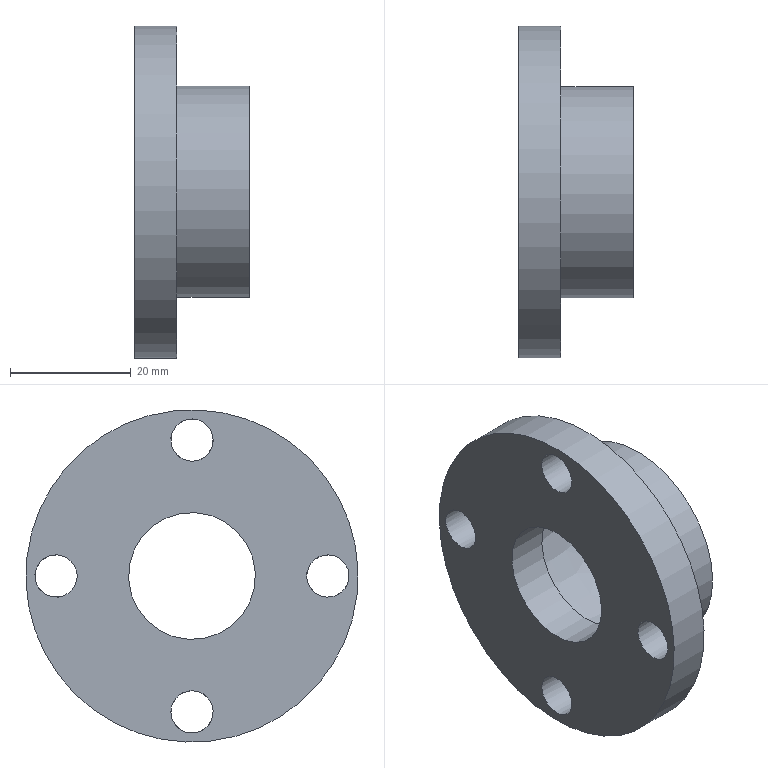Component | NX | BEARING_END_CAP_3 | 1 solid | 12 faces | box 19 x 55 x 55 mm | volume 16797 mm3 | cylinder 7 | plane 4 | cone 1 | commonest cylinder face diameters 7 x4 21 x1 35 x1 55 x1
STEP:
#1=CARTESIAN_POINT('',(0.,0.,0.));
#2=DIRECTION('',(0.,0.,1.));
#3=DIRECTION('',(1.,0.,0.));
#4=AXIS2_PLACEMENT_3D('',#1,#2,#3);
#5=CARTESIAN_POINT('',(407.689,-153.802,-1550.5));
#6=VERTEX_POINT('',#5);
#7=CARTESIAN_POINT('',(407.689,-152.777,-1548.025));
#8=VERTEX_POINT('',#7);
#9=CARTESIAN_POINT('',(407.689,-150.302,-1550.5));
#10=DIRECTION('',(-1.,0.,0.));
#11=DIRECTION('',(0.,-1.,0.));
#12=AXIS2_PLACEMENT_3D('',#9,#10,#11);
#13=CIRCLE('',#12,3.5);
#14=CARTESIAN_POINT('',(407.689,-169.747,-1553.555));
#15=DIRECTION('',(1.,0.,0.));
#16=DIRECTION('',(0.,0.7071,-0.7071));
#17=AXIS2_PLACEMENT_3D('',#14,#15,#16);
#18=PLANE('',#17);
#19=CARTESIAN_POINT('',(9.115,13.435));
#20=CARTESIAN_POINT('',(4.829,17.722));
#21=CARTESIAN_POINT('',(10.684,19.291));
#22=CARTESIAN_POINT('',(16.54,20.86));
#23=CARTESIAN_POINT('',(14.971,15.004));
#24=CARTESIAN_POINT('',(13.402,9.148));
#25=CARTESIAN_POINT('',(9.115,13.435));
#26=(BOUNDED_CURVE()B_SPLINE_CURVE(2,(#19,#20,#21,#22,#23,#24,#25),.UNSPECIFIED.,.T.,.F.)B_SPLINE_CURVE_WITH_KNOTS((1,2,2,2,2,1),(-2.094,0.,2.094,4.189,6.283,8.378),.UNSPECIFIED.)CURVE()GEOMETRIC_REPRESENTATION_ITEM()RATIONAL_B_SPLINE_CURVE((1.,0.5,1.,0.5,1.,0.5,1.))REPRESENTATION_ITEM(''));
#27=(GEOMETRIC_REPRESENTATION_CONTEXT(2)PARAMETRIC_REPRESENTATION_CONTEXT()REPRESENTATION_CONTEXT('',''));
#28=DEFINITIONAL_REPRESENTATION('',(#26),#27);
#29=PCURVE('',#18,#28);
#30=CARTESIAN_POINT('',(430.689,-150.302,-1550.5));
#31=DIRECTION('',(-1.,0.,0.));
#32=DIRECTION('',(0.,-0.7071,0.7071));
#33=AXIS2_PLACEMENT_3D('',#30,#31,#32);
#34=CYLINDRICAL_SURFACE('',#33,3.5);
#35=CARTESIAN_POINT('',(5.498,23.));
#36=DIRECTION('',(1.,0.));
#37=VECTOR('',#36,1.);
#38=LINE('',#35,#37);
#39=(GEOMETRIC_REPRESENTATION_CONTEXT(2)PARAMETRIC_REPRESENTATION_CONTEXT()REPRESENTATION_CONTEXT('',''));
#40=DEFINITIONAL_REPRESENTATION('',(#38),#39);
#41=PCURVE('',#34,#40);
#42=SURFACE_CURVE('',#13,(#29,#41),.PCURVE_S1.);
#43=EDGE_CURVE('',#6,#8,#42,.T.);
#44=ORIENTED_EDGE('',*,*,#43,.F.);
#45=CARTESIAN_POINT('',(407.689,-150.302,-1550.5));
#46=DIRECTION('',(-1.,0.,0.));
#47=DIRECTION('',(0.,-1.,0.));
#48=AXIS2_PLACEMENT_3D('',#45,#46,#47);
#49=CIRCLE('',#48,3.5);
#50=CARTESIAN_POINT('',(9.115,13.435));
#51=CARTESIAN_POINT('',(4.829,17.722));
#52=CARTESIAN_POINT('',(10.684,19.291));
#53=CARTESIAN_POINT('',(16.54,20.86));
#54=CARTESIAN_POINT('',(14.971,15.004));
#55=CARTESIAN_POINT('',(13.402,9.148));
#56=CARTESIAN_POINT('',(9.115,13.435));
#57=(BOUNDED_CURVE()B_SPLINE_CURVE(2,(#50,#51,#52,#53,#54,#55,#56),.UNSPECIFIED.,.T.,.F.)B_SPLINE_CURVE_WITH_KNOTS((1,2,2,2,2,1),(-2.094,0.,2.094,4.189,6.283,8.378),.UNSPECIFIED.)CURVE()GEOMETRIC_REPRESENTATION_ITEM()RATIONAL_B_SPLINE_CURVE((1.,0.5,1.,0.5,1.,0.5,1.))REPRESENTATION_ITEM(''));
#58=(GEOMETRIC_REPRESENTATION_CONTEXT(2)PARAMETRIC_REPRESENTATION_CONTEXT()REPRESENTATION_CONTEXT('',''));
#59=DEFINITIONAL_REPRESENTATION('',(#57),#58);
#60=PCURVE('',#18,#59);
#61=CARTESIAN_POINT('',(-0.7854,23.));
#62=DIRECTION('',(1.,0.));
#63=VECTOR('',#62,1.);
#64=LINE('',#61,#63);
#65=(GEOMETRIC_REPRESENTATION_CONTEXT(2)PARAMETRIC_REPRESENTATION_CONTEXT()REPRESENTATION_CONTEXT('',''));
#66=DEFINITIONAL_REPRESENTATION('',(#64),#65);
#67=PCURVE('',#34,#66);
#68=SURFACE_CURVE('',#49,(#60,#67),.PCURVE_S1.);
#69=EDGE_CURVE('',#8,#6,#68,.T.);
#70=ORIENTED_EDGE('',*,*,#69,.F.);
#71=EDGE_LOOP('',(#44,#70));
#72=FACE_BOUND('',#71,.T.);
#73=CARTESIAN_POINT('',(407.689,-172.802,-1576.5));
#74=VERTEX_POINT('',#73);
#75=CARTESIAN_POINT('',(407.689,-175.277,-1570.525));
#76=VERTEX_POINT('',#75);
#77=CARTESIAN_POINT('',(407.689,-172.802,-1573.));
#78=DIRECTION('',(-1.,0.,0.));
#79=DIRECTION('',(0.,0.,-1.));
#80=AXIS2_PLACEMENT_3D('',#77,#78,#79);
#81=CIRCLE('',#80,3.5);
#82=CARTESIAN_POINT('',(14.065,-18.385));
#83=CARTESIAN_POINT('',(9.778,-22.671));
#84=CARTESIAN_POINT('',(8.209,-16.816));
#85=CARTESIAN_POINT('',(6.64,-10.96));
#86=CARTESIAN_POINT('',(12.496,-12.529));
#87=CARTESIAN_POINT('',(18.352,-14.098));
#88=CARTESIAN_POINT('',(14.065,-18.385));
#89=(BOUNDED_CURVE()B_SPLINE_CURVE(2,(#82,#83,#84,#85,#86,#87,#88),.UNSPECIFIED.,.T.,.F.)B_SPLINE_CURVE_WITH_KNOTS((1,2,2,2,2,1),(-2.094,0.,2.094,4.189,6.283,8.378),.UNSPECIFIED.)CURVE()GEOMETRIC_REPRESENTATION_ITEM()RATIONAL_B_SPLINE_CURVE((1.,0.5,1.,0.5,1.,0.5,1.))REPRESENTATION_ITEM(''));
#90=(GEOMETRIC_REPRESENTATION_CONTEXT(2)PARAMETRIC_REPRESENTATION_CONTEXT()REPRESENTATION_CONTEXT('',''));
#91=DEFINITIONAL_REPRESENTATION('',(#89),#90);
#92=PCURVE('',#18,#91);
#93=CARTESIAN_POINT('',(430.689,-172.802,-1573.));
#94=DIRECTION('',(-1.,0.,0.));
#95=DIRECTION('',(0.,-0.7071,0.7071));
#96=AXIS2_PLACEMENT_3D('',#93,#94,#95);
#97=CYLINDRICAL_SURFACE('',#96,3.5);
#98=CARTESIAN_POINT('',(3.927,23.));
#99=DIRECTION('',(1.,0.));
#100=VECTOR('',#99,1.);
#101=LINE('',#98,#100);
#102=(GEOMETRIC_REPRESENTATION_CONTEXT(2)PARAMETRIC_REPRESENTATION_CONTEXT()REPRESENTATION_CONTEXT('',''));
#103=DEFINITIONAL_REPRESENTATION('',(#101),#102);
#104=PCURVE('',#97,#103);
#105=SURFACE_CURVE('',#81,(#92,#104),.PCURVE_S1.);
#106=EDGE_CURVE('',#74,#76,#105,.T.);
#107=ORIENTED_EDGE('',*,*,#106,.F.);
#108=CARTESIAN_POINT('',(407.689,-172.802,-1573.));
#109=DIRECTION('',(-1.,0.,0.));
#110=DIRECTION('',(0.,0.,-1.));
#111=AXIS2_PLACEMENT_3D('',#108,#109,#110);
#112=CIRCLE('',#111,3.5);
#113=CARTESIAN_POINT('',(14.065,-18.385));
#114=CARTESIAN_POINT('',(9.778,-22.671));
#115=CARTESIAN_POINT('',(8.209,-16.816));
#116=CARTESIAN_POINT('',(6.64,-10.96));
#117=CARTESIAN_POINT('',(12.496,-12.529));
#118=CARTESIAN_POINT('',(18.352,-14.098));
#119=CARTESIAN_POINT('',(14.065,-18.385));
#120=(BOUNDED_CURVE()B_SPLINE_CURVE(2,(#113,#114,#115,#116,#117,#118,#119),.UNSPECIFIED.,.T.,.F.)B_SPLINE_CURVE_WITH_KNOTS((1,2,2,2,2,1),(-2.094,0.,2.094,4.189,6.283,8.378),.UNSPECIFIED.)CURVE()GEOMETRIC_REPRESENTATION_ITEM()RATIONAL_B_SPLINE_CURVE((1.,0.5,1.,0.5,1.,0.5,1.))REPRESENTATION_ITEM(''));
#121=(GEOMETRIC_REPRESENTATION_CONTEXT(2)PARAMETRIC_REPRESENTATION_CONTEXT()REPRESENTATION_CONTEXT('',''));
#122=DEFINITIONAL_REPRESENTATION('',(#120),#121);
#123=PCURVE('',#18,#122);
#124=CARTESIAN_POINT('',(-2.356,23.));
#125=DIRECTION('',(1.,0.));
#126=VECTOR('',#125,1.);
#127=LINE('',#124,#126);
#128=(GEOMETRIC_REPRESENTATION_CONTEXT(2)PARAMETRIC_REPRESENTATION_CONTEXT()REPRESENTATION_CONTEXT('',''));
#129=DEFINITIONAL_REPRESENTATION('',(#127),#128);
#130=PCURVE('',#97,#129);
#131=SURFACE_CURVE('',#112,(#123,#130),.PCURVE_S1.);
#132=EDGE_CURVE('',#76,#74,#131,.T.);
#133=ORIENTED_EDGE('',*,*,#132,.F.);
#134=EDGE_LOOP('',(#107,#133));
#135=FACE_BOUND('',#134,.T.);
#136=CARTESIAN_POINT('',(407.689,-146.802,-1595.5));
#137=VERTEX_POINT('',#136);
#138=CARTESIAN_POINT('',(407.689,-152.777,-1593.025));
#139=VERTEX_POINT('',#138);
#140=CARTESIAN_POINT('',(407.689,-150.302,-1595.5));
#141=DIRECTION('',(-1.,0.,0.));
#142=DIRECTION('',(0.,1.,0.));
#143=AXIS2_PLACEMENT_3D('',#140,#141,#142);
#144=CIRCLE('',#143,3.5);
#145=CARTESIAN_POINT('',(45.885,-13.435));
#146=CARTESIAN_POINT('',(50.171,-17.722));
#147=CARTESIAN_POINT('',(44.316,-19.291));
#148=CARTESIAN_POINT('',(38.46,-20.86));
#149=CARTESIAN_POINT('',(40.029,-15.004));
#150=CARTESIAN_POINT('',(41.598,-9.148));
#151=CARTESIAN_POINT('',(45.885,-13.435));
#152=(BOUNDED_CURVE()B_SPLINE_CURVE(2,(#145,#146,#147,#148,#149,#150,#151),.UNSPECIFIED.,.T.,.F.)B_SPLINE_CURVE_WITH_KNOTS((1,2,2,2,2,1),(-2.094,0.,2.094,4.189,6.283,8.378),.UNSPECIFIED.)CURVE()GEOMETRIC_REPRESENTATION_ITEM()RATIONAL_B_SPLINE_CURVE((1.,0.5,1.,0.5,1.,0.5,1.))REPRESENTATION_ITEM(''));
#153=(GEOMETRIC_REPRESENTATION_CONTEXT(2)PARAMETRIC_REPRESENTATION_CONTEXT()REPRESENTATION_CONTEXT('',''));
#154=DEFINITIONAL_REPRESENTATION('',(#152),#153);
#155=PCURVE('',#18,#154);
#156=CARTESIAN_POINT('',(430.689,-150.302,-1595.5));
#157=DIRECTION('',(-1.,0.,0.));
#158=DIRECTION('',(0.,-0.7071,0.7071));
#159=AXIS2_PLACEMENT_3D('',#156,#157,#158);
#160=CYLINDRICAL_SURFACE('',#159,3.5);
#161=CARTESIAN_POINT('',(2.356,23.));
#162=DIRECTION('',(1.,0.));
#163=VECTOR('',#162,1.);
#164=LINE('',#161,#163);
#165=(GEOMETRIC_REPRESENTATION_CONTEXT(2)PARAMETRIC_REPRESENTATION_CONTEXT()REPRESENTATION_CONTEXT('',''));
#166=DEFINITIONAL_REPRESENTATION('',(#164),#165);
#167=PCURVE('',#160,#166);
#168=SURFACE_CURVE('',#144,(#155,#167),.PCURVE_S1.);
#169=EDGE_CURVE('',#137,#139,#168,.T.);
#170=ORIENTED_EDGE('',*,*,#169,.F.);
#171=CARTESIAN_POINT('',(407.689,-150.302,-1595.5));
#172=DIRECTION('',(-1.,0.,0.));
#173=DIRECTION('',(0.,1.,0.));
#174=AXIS2_PLACEMENT_3D('',#171,#172,#173);
#175=CIRCLE('',#174,3.5);
#176=CARTESIAN_POINT('',(45.885,-13.435));
#177=CARTESIAN_POINT('',(50.171,-17.722));
#178=CARTESIAN_POINT('',(44.316,-19.291));
#179=CARTESIAN_POINT('',(38.46,-20.86));
#180=CARTESIAN_POINT('',(40.029,-15.004));
#181=CARTESIAN_POINT('',(41.598,-9.148));
#182=CARTESIAN_POINT('',(45.885,-13.435));
#183=(BOUNDED_CURVE()B_SPLINE_CURVE(2,(#176,#177,#178,#179,#180,#181,#182),.UNSPECIFIED.,.T.,.F.)B_SPLINE_CURVE_WITH_KNOTS((1,2,2,2,2,1),(-2.094,0.,2.094,4.189,6.283,8.378),.UNSPECIFIED.)CURVE()GEOMETRIC_REPRESENTATION_ITEM()RATIONAL_B_SPLINE_CURVE((1.,0.5,1.,0.5,1.,0.5,1.))REPRESENTATION_ITEM(''));
#184=(GEOMETRIC_REPRESENTATION_CONTEXT(2)PARAMETRIC_REPRESENTATION_CONTEXT()REPRESENTATION_CONTEXT('',''));
#185=DEFINITIONAL_REPRESENTATION('',(#183),#184);
#186=PCURVE('',#18,#185);
#187=CARTESIAN_POINT('',(-3.927,23.));
#188=DIRECTION('',(1.,0.));
#189=VECTOR('',#188,1.);
#190=LINE('',#187,#189);
#191=(GEOMETRIC_REPRESENTATION_CONTEXT(2)PARAMETRIC_REPRESENTATION_CONTEXT()REPRESENTATION_CONTEXT('',''));
#192=DEFINITIONAL_REPRESENTATION('',(#190),#191);
#193=PCURVE('',#160,#192);
#194=SURFACE_CURVE('',#175,(#186,#193),.PCURVE_S1.);
#195=EDGE_CURVE('',#139,#137,#194,.T.);
#196=ORIENTED_EDGE('',*,*,#195,.F.);
#197=EDGE_LOOP('',(#170,#196));
#198=FACE_BOUND('',#197,.T.);
#199=CARTESIAN_POINT('',(407.689,-127.802,-1569.5));
#200=VERTEX_POINT('',#199);
#201=CARTESIAN_POINT('',(407.689,-130.277,-1570.525));
#202=VERTEX_POINT('',#201);
#203=CARTESIAN_POINT('',(407.689,-127.802,-1573.));
#204=DIRECTION('',(-1.,0.,0.));
#205=DIRECTION('',(0.,0.,1.));
#206=AXIS2_PLACEMENT_3D('',#203,#204,#205);
#207=CIRCLE('',#206,3.5);
#208=CARTESIAN_POINT('',(40.935,18.385));
#209=CARTESIAN_POINT('',(45.222,22.671));
#210=CARTESIAN_POINT('',(46.791,16.816));
#211=CARTESIAN_POINT('',(48.36,10.96));
#212=CARTESIAN_POINT('',(42.504,12.529));
#213=CARTESIAN_POINT('',(36.648,14.098));
#214=CARTESIAN_POINT('',(40.935,18.385));
#215=(BOUNDED_CURVE()B_SPLINE_CURVE(2,(#208,#209,#210,#211,#212,#213,#214),.UNSPECIFIED.,.T.,.F.)B_SPLINE_CURVE_WITH_KNOTS((1,2,2,2,2,1),(-2.094,0.,2.094,4.189,6.283,8.378),.UNSPECIFIED.)CURVE()GEOMETRIC_REPRESENTATION_ITEM()RATIONAL_B_SPLINE_CURVE((1.,0.5,1.,0.5,1.,0.5,1.))REPRESENTATION_ITEM(''));
#216=(GEOMETRIC_REPRESENTATION_CONTEXT(2)PARAMETRIC_REPRESENTATION_CONTEXT()REPRESENTATION_CONTEXT('',''));
#217=DEFINITIONAL_REPRESENTATION('',(#215),#216);
#218=PCURVE('',#18,#217);
#219=CARTESIAN_POINT('',(430.689,-127.802,-1573.));
#220=DIRECTION('',(-1.,0.,0.));
#221=DIRECTION('',(0.,-0.7071,0.7071));
#222=AXIS2_PLACEMENT_3D('',#219,#220,#221);
#223=CYLINDRICAL_SURFACE('',#222,3.5);
#224=CARTESIAN_POINT('',(0.7854,23.));
#225=DIRECTION('',(1.,0.));
#226=VECTOR('',#225,1.);
#227=LINE('',#224,#226);
#228=(GEOMETRIC_REPRESENTATION_CONTEXT(2)PARAMETRIC_REPRESENTATION_CONTEXT()REPRESENTATION_CONTEXT('',''));
#229=DEFINITIONAL_REPRESENTATION('',(#227),#228);
#230=PCURVE('',#223,#229);
#231=SURFACE_CURVE('',#207,(#218,#230),.PCURVE_S1.);
#232=EDGE_CURVE('',#200,#202,#231,.T.);
#233=ORIENTED_EDGE('',*,*,#232,.F.);
#234=CARTESIAN_POINT('',(407.689,-127.802,-1573.));
#235=DIRECTION('',(-1.,0.,0.));
#236=DIRECTION('',(0.,0.,1.));
#237=AXIS2_PLACEMENT_3D('',#234,#235,#236);
#238=CIRCLE('',#237,3.5);
#239=CARTESIAN_POINT('',(40.935,18.385));
#240=CARTESIAN_POINT('',(45.222,22.671));
#241=CARTESIAN_POINT('',(46.791,16.816));
#242=CARTESIAN_POINT('',(48.36,10.96));
#243=CARTESIAN_POINT('',(42.504,12.529));
#244=CARTESIAN_POINT('',(36.648,14.098));
#245=CARTESIAN_POINT('',(40.935,18.385));
#246=(BOUNDED_CURVE()B_SPLINE_CURVE(2,(#239,#240,#241,#242,#243,#244,#245),.UNSPECIFIED.,.T.,.F.)B_SPLINE_CURVE_WITH_KNOTS((1,2,2,2,2,1),(-2.094,0.,2.094,4.189,6.283,8.378),.UNSPECIFIED.)CURVE()GEOMETRIC_REPRESENTATION_ITEM()RATIONAL_B_SPLINE_CURVE((1.,0.5,1.,0.5,1.,0.5,1.))REPRESENTATION_ITEM(''));
#247=(GEOMETRIC_REPRESENTATION_CONTEXT(2)PARAMETRIC_REPRESENTATION_CONTEXT()REPRESENTATION_CONTEXT('',''));
#248=DEFINITIONAL_REPRESENTATION('',(#246),#247);
#249=PCURVE('',#18,#248);
#250=CARTESIAN_POINT('',(-5.498,23.));
#251=DIRECTION('',(1.,0.));
#252=VECTOR('',#251,1.);
#253=LINE('',#250,#252);
#254=(GEOMETRIC_REPRESENTATION_CONTEXT(2)PARAMETRIC_REPRESENTATION_CONTEXT()REPRESENTATION_CONTEXT('',''));
#255=DEFINITIONAL_REPRESENTATION('',(#253),#254);
#256=PCURVE('',#223,#255);
#257=SURFACE_CURVE('',#238,(#249,#256),.PCURVE_S1.);
#258=EDGE_CURVE('',#202,#200,#257,.T.);
#259=ORIENTED_EDGE('',*,*,#258,.F.);
#260=EDGE_LOOP('',(#233,#259));
#261=FACE_BOUND('',#260,.T.);
#262=CARTESIAN_POINT('',(407.689,-157.726,-1565.575));
#263=VERTEX_POINT('',#262);
#264=CARTESIAN_POINT('',(407.689,-150.302,-1573.));
#265=DIRECTION('',(-1.,0.,0.));
#266=DIRECTION('',(0.,-0.7071,0.7071));
#267=AXIS2_PLACEMENT_3D('',#264,#265,#266);
#268=CIRCLE('',#267,10.5);
#269=CARTESIAN_POINT('',(17.,0.));
#270=CARTESIAN_POINT('',(17.,18.187));
#271=CARTESIAN_POINT('',(32.75,9.093));
#272=CARTESIAN_POINT('',(48.5,0.));
#273=CARTESIAN_POINT('',(32.75,-9.093));
#274=CARTESIAN_POINT('',(17.,-18.187));
#275=CARTESIAN_POINT('',(17.,0.));
#276=(BOUNDED_CURVE()B_SPLINE_CURVE(2,(#269,#270,#271,#272,#273,#274,#275),.UNSPECIFIED.,.T.,.F.)B_SPLINE_CURVE_WITH_KNOTS((1,2,2,2,2,1),(-2.094,0.,2.094,4.189,6.283,8.378),.UNSPECIFIED.)CURVE()GEOMETRIC_REPRESENTATION_ITEM()RATIONAL_B_SPLINE_CURVE((1.,0.5,1.,0.5,1.,0.5,1.))REPRESENTATION_ITEM(''));
#277=(GEOMETRIC_REPRESENTATION_CONTEXT(2)PARAMETRIC_REPRESENTATION_CONTEXT()REPRESENTATION_CONTEXT('',''));
#278=DEFINITIONAL_REPRESENTATION('',(#276),#277);
#279=PCURVE('',#18,#278);
#280=CARTESIAN_POINT('',(407.689,-150.302,-1573.));
#281=DIRECTION('',(-1.,0.,0.));
#282=DIRECTION('',(0.,-0.7071,0.7071));
#283=AXIS2_PLACEMENT_3D('',#280,#281,#282);
#284=CYLINDRICAL_SURFACE('',#283,10.5);
#285=CARTESIAN_POINT('',(0.,0.));
#286=DIRECTION('',(1.,0.));
#287=VECTOR('',#286,1.);
#288=LINE('',#285,#287);
#289=(GEOMETRIC_REPRESENTATION_CONTEXT(2)PARAMETRIC_REPRESENTATION_CONTEXT()REPRESENTATION_CONTEXT('',''));
#290=DEFINITIONAL_REPRESENTATION('',(#288),#289);
#291=PCURVE('',#284,#290);
#292=SURFACE_CURVE('',#268,(#279,#291),.PCURVE_S1.);
#293=EDGE_CURVE('',#263,#263,#292,.T.);
#294=ORIENTED_EDGE('',*,*,#293,.F.);
#295=EDGE_LOOP('',(#294));
#296=FACE_BOUND('',#295,.T.);
#297=CARTESIAN_POINT('',(407.689,-169.747,-1553.555));
#298=VERTEX_POINT('',#297);
#299=CARTESIAN_POINT('',(407.689,-150.302,-1573.));
#300=DIRECTION('',(-1.,0.,0.));
#301=DIRECTION('',(0.,-0.7071,0.7071));
#302=AXIS2_PLACEMENT_3D('',#299,#300,#301);
#303=CIRCLE('',#302,27.5);
#304=CARTESIAN_POINT('',(-0.,-0.));
#305=CARTESIAN_POINT('',(-0.,47.631));
#306=CARTESIAN_POINT('',(41.25,23.816));
#307=CARTESIAN_POINT('',(82.5,0.));
#308=CARTESIAN_POINT('',(41.25,-23.816));
#309=CARTESIAN_POINT('',(0.,-47.631));
#310=CARTESIAN_POINT('',(-0.,-0.));
#311=(BOUNDED_CURVE()B_SPLINE_CURVE(2,(#304,#305,#306,#307,#308,#309,#310),.UNSPECIFIED.,.T.,.F.)B_SPLINE_CURVE_WITH_KNOTS((1,2,2,2,2,1),(-2.094,0.,2.094,4.189,6.283,8.378),.UNSPECIFIED.)CURVE()GEOMETRIC_REPRESENTATION_ITEM()RATIONAL_B_SPLINE_CURVE((1.,0.5,1.,0.5,1.,0.5,1.))REPRESENTATION_ITEM(''));
#312=(GEOMETRIC_REPRESENTATION_CONTEXT(2)PARAMETRIC_REPRESENTATION_CONTEXT()REPRESENTATION_CONTEXT('',''));
#313=DEFINITIONAL_REPRESENTATION('',(#311),#312);
#314=PCURVE('',#18,#313);
#315=CARTESIAN_POINT('',(407.689,-150.302,-1573.));
#316=DIRECTION('',(-1.,0.,0.));
#317=DIRECTION('',(0.,-0.7071,0.7071));
#318=AXIS2_PLACEMENT_3D('',#315,#316,#317);
#319=CYLINDRICAL_SURFACE('',#318,27.5);
#320=CARTESIAN_POINT('',(0.,0.));
#321=DIRECTION('',(1.,0.));
#322=VECTOR('',#321,1.);
#323=LINE('',#320,#322);
#324=(GEOMETRIC_REPRESENTATION_CONTEXT(2)PARAMETRIC_REPRESENTATION_CONTEXT()REPRESENTATION_CONTEXT('',''));
#325=DEFINITIONAL_REPRESENTATION('',(#323),#324);
#326=PCURVE('',#319,#325);
#327=SURFACE_CURVE('',#303,(#314,#326),.PCURVE_S1.);
#328=EDGE_CURVE('',#298,#298,#327,.T.);
#329=ORIENTED_EDGE('',*,*,#328,.T.);
#330=EDGE_LOOP('',(#329));
#331=FACE_BOUND('',#330,.T.);
#332=ADVANCED_FACE('',(#72,#135,#198,#261,#296,#331),#18,.F.);
#333=CARTESIAN_POINT('',(414.689,-157.726,-1565.575));
#334=VERTEX_POINT('',#333);
#335=CARTESIAN_POINT('',(414.689,-150.302,-1573.));
#336=DIRECTION('',(-1.,0.,0.));
#337=DIRECTION('',(0.,-0.7071,0.7071));
#338=AXIS2_PLACEMENT_3D('',#335,#336,#337);
#339=CIRCLE('',#338,10.5);
#340=CARTESIAN_POINT('',(0.,-7.));
#341=DIRECTION('',(1.,0.));
#342=VECTOR('',#341,1.);
#343=LINE('',#340,#342);
#344=(GEOMETRIC_REPRESENTATION_CONTEXT(2)PARAMETRIC_REPRESENTATION_CONTEXT()REPRESENTATION_CONTEXT('',''));
#345=DEFINITIONAL_REPRESENTATION('',(#343),#344);
#346=PCURVE('',#284,#345);
#347=CARTESIAN_POINT('',(414.689,-157.726,-1565.575));
#348=DIRECTION('',(-1.,0.,0.));
#349=DIRECTION('',(0.,-0.7071,0.7071));
#350=AXIS2_PLACEMENT_3D('',#347,#348,#349);
#351=PLANE('',#350);
#352=CARTESIAN_POINT('',(-10.5,-0.));
#353=DIRECTION('',(1.,-0.));
#354=AXIS2_PLACEMENT_2D('',#352,#353);
#355=CIRCLE('',#354,10.5);
#356=(GEOMETRIC_REPRESENTATION_CONTEXT(2)PARAMETRIC_REPRESENTATION_CONTEXT()REPRESENTATION_CONTEXT('',''));
#357=DEFINITIONAL_REPRESENTATION('',(#355),#356);
#358=PCURVE('',#351,#357);
#359=SURFACE_CURVE('',#339,(#346,#358),.PCURVE_S1.);
#360=EDGE_CURVE('',#334,#334,#359,.T.);
#361=ORIENTED_EDGE('',*,*,#360,.T.);
#362=CARTESIAN_POINT('',(414.689,-157.726,-1565.575));
#363=CARTESIAN_POINT('',(407.689,-157.726,-1565.575));
#364=B_SPLINE_CURVE_WITH_KNOTS('',1,(#362,#363),.UNSPECIFIED.,.F.,.F.,(2,2),(-7.,0.),.PIECEWISE_BEZIER_KNOTS.);
#365=CARTESIAN_POINT('',(6.283,0.));
#366=DIRECTION('',(0.,1.));
#367=VECTOR('',#366,1.);
#368=LINE('',#365,#367);
#369=(GEOMETRIC_REPRESENTATION_CONTEXT(2)PARAMETRIC_REPRESENTATION_CONTEXT()REPRESENTATION_CONTEXT('',''));
#370=DEFINITIONAL_REPRESENTATION('',(#368),#369);
#371=PCURVE('',#284,#370);
#372=CARTESIAN_POINT('',(0.,0.));
#373=DIRECTION('',(0.,1.));
#374=VECTOR('',#373,1.);
#375=LINE('',#372,#374);
#376=(GEOMETRIC_REPRESENTATION_CONTEXT(2)PARAMETRIC_REPRESENTATION_CONTEXT()REPRESENTATION_CONTEXT('',''));
#377=DEFINITIONAL_REPRESENTATION('',(#375),#376);
#378=PCURVE('',#284,#377);
#379=SEAM_CURVE('',#364,(#371,#378),.PCURVE_S1.);
#380=EDGE_CURVE('',#334,#263,#379,.T.);
#381=ORIENTED_EDGE('',*,*,#380,.T.);
#382=ORIENTED_EDGE('',*,*,#293,.F.);
#383=ORIENTED_EDGE('',*,*,#380,.F.);
#384=EDGE_LOOP('',(#361,#381,#382,#383));
#385=FACE_BOUND('',#384,.F.);
#386=ADVANCED_FACE('',(#385),#284,.F.);
#387=CARTESIAN_POINT('',(414.689,-159.766,-1563.536));
#388=VERTEX_POINT('',#387);
#389=CARTESIAN_POINT('',(414.689,-150.302,-1573.));
#390=DIRECTION('',(-1.,0.,0.));
#391=DIRECTION('',(0.,-0.7071,0.7071));
#392=AXIS2_PLACEMENT_3D('',#389,#390,#391);
#393=CIRCLE('',#392,13.384);
#394=CARTESIAN_POINT('',(-10.5,-0.));
#395=DIRECTION('',(1.,0.));
#396=AXIS2_PLACEMENT_2D('',#394,#395);
#397=CIRCLE('',#396,13.384);
#398=(GEOMETRIC_REPRESENTATION_CONTEXT(2)PARAMETRIC_REPRESENTATION_CONTEXT()REPRESENTATION_CONTEXT('',''));
#399=DEFINITIONAL_REPRESENTATION('',(#397),#398);
#400=PCURVE('',#351,#399);
#401=CARTESIAN_POINT('',(414.689,-150.302,-1573.));
#402=DIRECTION('',(1.,0.,0.));
#403=DIRECTION('',(0.,0.7071,-0.7071));
#404=AXIS2_PLACEMENT_3D('',#401,#402,#403);
#405=CONICAL_SURFACE('',#404,13.384,0.1745);
#406=CARTESIAN_POINT('',(9.425,-0.));
#407=DIRECTION('',(-1.,0.));
#408=VECTOR('',#407,1.);
#409=LINE('',#406,#408);
#410=(GEOMETRIC_REPRESENTATION_CONTEXT(2)PARAMETRIC_REPRESENTATION_CONTEXT()REPRESENTATION_CONTEXT('',''));
#411=DEFINITIONAL_REPRESENTATION('',(#409),#410);
#412=PCURVE('',#405,#411);
#413=SURFACE_CURVE('',#393,(#400,#412),.PCURVE_S1.);
#414=EDGE_CURVE('',#388,#388,#413,.T.);
#415=ORIENTED_EDGE('',*,*,#414,.F.);
#416=EDGE_LOOP('',(#415));
#417=FACE_BOUND('',#416,.T.);
#418=ORIENTED_EDGE('',*,*,#360,.T.);
#419=EDGE_LOOP('',(#418));
#420=FACE_BOUND('',#419,.T.);
#421=ADVANCED_FACE('',(#417,#420),#351,.F.);
#422=CARTESIAN_POINT('',(426.689,-161.262,-1562.04));
#423=VERTEX_POINT('',#422);
#424=CARTESIAN_POINT('',(426.689,-150.302,-1573.));
#425=DIRECTION('',(-1.,0.,0.));
#426=DIRECTION('',(0.,-0.7071,0.7071));
#427=AXIS2_PLACEMENT_3D('',#424,#425,#426);
#428=CIRCLE('',#427,15.5);
#429=CARTESIAN_POINT('',(9.425,12.));
#430=DIRECTION('',(-1.,0.));
#431=VECTOR('',#430,1.);
#432=LINE('',#429,#431);
#433=(GEOMETRIC_REPRESENTATION_CONTEXT(2)PARAMETRIC_REPRESENTATION_CONTEXT()REPRESENTATION_CONTEXT('',''));
#434=DEFINITIONAL_REPRESENTATION('',(#432),#433);
#435=PCURVE('',#405,#434);
#436=CARTESIAN_POINT('',(426.689,-161.262,-1562.04));
#437=DIRECTION('',(-1.,0.,0.));
#438=DIRECTION('',(0.,-0.7071,0.7071));
#439=AXIS2_PLACEMENT_3D('',#436,#437,#438);
#440=PLANE('',#439);
#441=CARTESIAN_POINT('',(-15.5,0.));
#442=DIRECTION('',(1.,-0.));
#443=AXIS2_PLACEMENT_2D('',#441,#442);
#444=CIRCLE('',#443,15.5);
#445=(GEOMETRIC_REPRESENTATION_CONTEXT(2)PARAMETRIC_REPRESENTATION_CONTEXT()REPRESENTATION_CONTEXT('',''));
#446=DEFINITIONAL_REPRESENTATION('',(#444),#445);
#447=PCURVE('',#440,#446);
#448=SURFACE_CURVE('',#428,(#435,#447),.PCURVE_S1.);
#449=EDGE_CURVE('',#423,#423,#448,.T.);
#450=ORIENTED_EDGE('',*,*,#449,.T.);
#451=CARTESIAN_POINT('',(414.689,-159.766,-1563.536));
#452=CARTESIAN_POINT('',(426.689,-161.262,-1562.04));
#453=B_SPLINE_CURVE_WITH_KNOTS('',1,(#451,#452),.UNSPECIFIED.,.F.,.F.,(2,2),(-0.,12.185),.PIECEWISE_BEZIER_KNOTS.);
#454=CARTESIAN_POINT('',(3.142,0.));
#455=DIRECTION('',(0.,1.));
#456=VECTOR('',#455,1.);
#457=LINE('',#454,#456);
#458=(GEOMETRIC_REPRESENTATION_CONTEXT(2)PARAMETRIC_REPRESENTATION_CONTEXT()REPRESENTATION_CONTEXT('',''));
#459=DEFINITIONAL_REPRESENTATION('',(#457),#458);
#460=PCURVE('',#405,#459);
#461=CARTESIAN_POINT('',(9.425,0.));
#462=DIRECTION('',(0.,1.));
#463=VECTOR('',#462,1.);
#464=LINE('',#461,#463);
#465=(GEOMETRIC_REPRESENTATION_CONTEXT(2)PARAMETRIC_REPRESENTATION_CONTEXT()REPRESENTATION_CONTEXT('',''));
#466=DEFINITIONAL_REPRESENTATION('',(#464),#465);
#467=PCURVE('',#405,#466);
#468=SEAM_CURVE('',#453,(#460,#467),.PCURVE_S1.);
#469=EDGE_CURVE('',#388,#423,#468,.T.);
#470=ORIENTED_EDGE('',*,*,#469,.F.);
#471=ORIENTED_EDGE('',*,*,#414,.F.);
#472=ORIENTED_EDGE('',*,*,#469,.T.);
#473=EDGE_LOOP('',(#450,#470,#471,#472));
#474=FACE_BOUND('',#473,.F.);
#475=ADVANCED_FACE('',(#474),#405,.F.);
#476=CARTESIAN_POINT('',(426.689,-162.676,-1560.626));
#477=VERTEX_POINT('',#476);
#478=CARTESIAN_POINT('',(426.689,-150.302,-1573.));
#479=DIRECTION('',(-1.,0.,0.));
#480=DIRECTION('',(0.,-0.7071,0.7071));
#481=AXIS2_PLACEMENT_3D('',#478,#479,#480);
#482=CIRCLE('',#481,17.5);
#483=CARTESIAN_POINT('',(-15.5,0.));
#484=DIRECTION('',(1.,0.));
#485=AXIS2_PLACEMENT_2D('',#483,#484);
#486=CIRCLE('',#485,17.5);
#487=(GEOMETRIC_REPRESENTATION_CONTEXT(2)PARAMETRIC_REPRESENTATION_CONTEXT()REPRESENTATION_CONTEXT('',''));
#488=DEFINITIONAL_REPRESENTATION('',(#486),#487);
#489=PCURVE('',#440,#488);
#490=CARTESIAN_POINT('',(407.689,-150.302,-1573.));
#491=DIRECTION('',(-1.,0.,0.));
#492=DIRECTION('',(0.,-0.7071,0.7071));
#493=AXIS2_PLACEMENT_3D('',#490,#491,#492);
#494=CYLINDRICAL_SURFACE('',#493,17.5);
#495=CARTESIAN_POINT('',(0.,-19.));
#496=DIRECTION('',(1.,0.));
#497=VECTOR('',#496,1.);
#498=LINE('',#495,#497);
#499=(GEOMETRIC_REPRESENTATION_CONTEXT(2)PARAMETRIC_REPRESENTATION_CONTEXT()REPRESENTATION_CONTEXT('',''));
#500=DEFINITIONAL_REPRESENTATION('',(#498),#499);
#501=PCURVE('',#494,#500);
#502=SURFACE_CURVE('',#482,(#489,#501),.PCURVE_S1.);
#503=EDGE_CURVE('',#477,#477,#502,.T.);
#504=ORIENTED_EDGE('',*,*,#503,.F.);
#505=EDGE_LOOP('',(#504));
#506=FACE_BOUND('',#505,.T.);
#507=ORIENTED_EDGE('',*,*,#449,.T.);
#508=EDGE_LOOP('',(#507));
#509=FACE_BOUND('',#508,.T.);
#510=ADVANCED_FACE('',(#506,#509),#440,.F.);
#511=CARTESIAN_POINT('',(414.689,-162.676,-1560.626));
#512=VERTEX_POINT('',#511);
#513=CARTESIAN_POINT('',(414.689,-150.302,-1573.));
#514=DIRECTION('',(-1.,0.,0.));
#515=DIRECTION('',(0.,-0.7071,0.7071));
#516=AXIS2_PLACEMENT_3D('',#513,#514,#515);
#517=CIRCLE('',#516,17.5);
#518=CARTESIAN_POINT('',(0.,-7.));
#519=DIRECTION('',(1.,0.));
#520=VECTOR('',#519,1.);
#521=LINE('',#518,#520);
#522=(GEOMETRIC_REPRESENTATION_CONTEXT(2)PARAMETRIC_REPRESENTATION_CONTEXT()REPRESENTATION_CONTEXT('',''));
#523=DEFINITIONAL_REPRESENTATION('',(#521),#522);
#524=PCURVE('',#494,#523);
#525=CARTESIAN_POINT('',(414.689,-162.676,-1560.626));
#526=DIRECTION('',(-1.,0.,0.));
#527=DIRECTION('',(0.,-0.7071,0.7071));
#528=AXIS2_PLACEMENT_3D('',#525,#526,#527);
#529=PLANE('',#528);
#530=CARTESIAN_POINT('',(-17.5,0.));
#531=DIRECTION('',(1.,0.));
#532=AXIS2_PLACEMENT_2D('',#530,#531);
#533=CIRCLE('',#532,17.5);
#534=(GEOMETRIC_REPRESENTATION_CONTEXT(2)PARAMETRIC_REPRESENTATION_CONTEXT()REPRESENTATION_CONTEXT('',''));
#535=DEFINITIONAL_REPRESENTATION('',(#533),#534);
#536=PCURVE('',#529,#535);
#537=SURFACE_CURVE('',#517,(#524,#536),.PCURVE_S1.);
#538=EDGE_CURVE('',#512,#512,#537,.T.);
#539=ORIENTED_EDGE('',*,*,#538,.F.);
#540=CARTESIAN_POINT('',(426.689,-162.676,-1560.626));
#541=CARTESIAN_POINT('',(414.689,-162.676,-1560.626));
#542=B_SPLINE_CURVE_WITH_KNOTS('',1,(#540,#541),.UNSPECIFIED.,.F.,.F.,(2,2),(-19.,-7.),.PIECEWISE_BEZIER_KNOTS.);
#543=CARTESIAN_POINT('',(0.,0.));
#544=DIRECTION('',(0.,1.));
#545=VECTOR('',#544,1.);
#546=LINE('',#543,#545);
#547=(GEOMETRIC_REPRESENTATION_CONTEXT(2)PARAMETRIC_REPRESENTATION_CONTEXT()REPRESENTATION_CONTEXT('',''));
#548=DEFINITIONAL_REPRESENTATION('',(#546),#547);
#549=PCURVE('',#494,#548);
#550=CARTESIAN_POINT('',(6.283,0.));
#551=DIRECTION('',(0.,1.));
#552=VECTOR('',#551,1.);
#553=LINE('',#550,#552);
#554=(GEOMETRIC_REPRESENTATION_CONTEXT(2)PARAMETRIC_REPRESENTATION_CONTEXT()REPRESENTATION_CONTEXT('',''));
#555=DEFINITIONAL_REPRESENTATION('',(#553),#554);
#556=PCURVE('',#494,#555);
#557=SEAM_CURVE('',#542,(#549,#556),.PCURVE_S1.);
#558=EDGE_CURVE('',#477,#512,#557,.T.);
#559=ORIENTED_EDGE('',*,*,#558,.F.);
#560=ORIENTED_EDGE('',*,*,#503,.T.);
#561=ORIENTED_EDGE('',*,*,#558,.T.);
#562=EDGE_LOOP('',(#539,#559,#560,#561));
#563=FACE_BOUND('',#562,.T.);
#564=ADVANCED_FACE('',(#563),#494,.T.);
#565=CARTESIAN_POINT('',(414.689,-152.777,-1548.025));
#566=VERTEX_POINT('',#565);
#567=CARTESIAN_POINT('',(414.689,-150.302,-1550.5));
#568=DIRECTION('',(-1.,0.,0.));
#569=DIRECTION('',(0.,-0.7071,0.7071));
#570=AXIS2_PLACEMENT_3D('',#567,#568,#569);
#571=CIRCLE('',#570,3.5);
#572=CARTESIAN_POINT('',(-1.59,15.91));
#573=DIRECTION('',(1.,-0.));
#574=AXIS2_PLACEMENT_2D('',#572,#573);
#575=CIRCLE('',#574,3.5);
#576=(GEOMETRIC_REPRESENTATION_CONTEXT(2)PARAMETRIC_REPRESENTATION_CONTEXT()REPRESENTATION_CONTEXT('',''));
#577=DEFINITIONAL_REPRESENTATION('',(#575),#576);
#578=PCURVE('',#529,#577);
#579=CARTESIAN_POINT('',(0.,16.));
#580=DIRECTION('',(1.,0.));
#581=VECTOR('',#580,1.);
#582=LINE('',#579,#581);
#583=(GEOMETRIC_REPRESENTATION_CONTEXT(2)PARAMETRIC_REPRESENTATION_CONTEXT()REPRESENTATION_CONTEXT('',''));
#584=DEFINITIONAL_REPRESENTATION('',(#582),#583);
#585=PCURVE('',#34,#584);
#586=SURFACE_CURVE('',#571,(#578,#585),.PCURVE_S1.);
#587=EDGE_CURVE('',#566,#566,#586,.T.);
#588=ORIENTED_EDGE('',*,*,#587,.T.);
#589=EDGE_LOOP('',(#588));
#590=FACE_BOUND('',#589,.T.);
#591=CARTESIAN_POINT('',(414.689,-175.277,-1570.525));
#592=VERTEX_POINT('',#591);
#593=CARTESIAN_POINT('',(414.689,-172.802,-1573.));
#594=DIRECTION('',(-1.,0.,0.));
#595=DIRECTION('',(0.,-0.7071,0.7071));
#596=AXIS2_PLACEMENT_3D('',#593,#594,#595);
#597=CIRCLE('',#596,3.5);
#598=CARTESIAN_POINT('',(-1.59,-15.91));
#599=DIRECTION('',(1.,-0.));
#600=AXIS2_PLACEMENT_2D('',#598,#599);
#601=CIRCLE('',#600,3.5);
#602=(GEOMETRIC_REPRESENTATION_CONTEXT(2)PARAMETRIC_REPRESENTATION_CONTEXT()REPRESENTATION_CONTEXT('',''));
#603=DEFINITIONAL_REPRESENTATION('',(#601),#602);
#604=PCURVE('',#529,#603);
#605=CARTESIAN_POINT('',(0.,16.));
#606=DIRECTION('',(1.,0.));
#607=VECTOR('',#606,1.);
#608=LINE('',#605,#607);
#609=(GEOMETRIC_REPRESENTATION_CONTEXT(2)PARAMETRIC_REPRESENTATION_CONTEXT()REPRESENTATION_CONTEXT('',''));
#610=DEFINITIONAL_REPRESENTATION('',(#608),#609);
#611=PCURVE('',#97,#610);
#612=SURFACE_CURVE('',#597,(#604,#611),.PCURVE_S1.);
#613=EDGE_CURVE('',#592,#592,#612,.T.);
#614=ORIENTED_EDGE('',*,*,#613,.T.);
#615=EDGE_LOOP('',(#614));
#616=FACE_BOUND('',#615,.T.);
#617=CARTESIAN_POINT('',(414.689,-152.777,-1593.025));
#618=VERTEX_POINT('',#617);
#619=CARTESIAN_POINT('',(414.689,-150.302,-1595.5));
#620=DIRECTION('',(-1.,0.,0.));
#621=DIRECTION('',(0.,-0.7071,0.7071));
#622=AXIS2_PLACEMENT_3D('',#619,#620,#621);
#623=CIRCLE('',#622,3.5);
#624=CARTESIAN_POINT('',(-33.41,-15.91));
#625=DIRECTION('',(1.,-0.));
#626=AXIS2_PLACEMENT_2D('',#624,#625);
#627=CIRCLE('',#626,3.5);
#628=(GEOMETRIC_REPRESENTATION_CONTEXT(2)PARAMETRIC_REPRESENTATION_CONTEXT()REPRESENTATION_CONTEXT('',''));
#629=DEFINITIONAL_REPRESENTATION('',(#627),#628);
#630=PCURVE('',#529,#629);
#631=CARTESIAN_POINT('',(0.,16.));
#632=DIRECTION('',(1.,0.));
#633=VECTOR('',#632,1.);
#634=LINE('',#631,#633);
#635=(GEOMETRIC_REPRESENTATION_CONTEXT(2)PARAMETRIC_REPRESENTATION_CONTEXT()REPRESENTATION_CONTEXT('',''));
#636=DEFINITIONAL_REPRESENTATION('',(#634),#635);
#637=PCURVE('',#160,#636);
#638=SURFACE_CURVE('',#623,(#630,#637),.PCURVE_S1.);
#639=EDGE_CURVE('',#618,#618,#638,.T.);
#640=ORIENTED_EDGE('',*,*,#639,.T.);
#641=EDGE_LOOP('',(#640));
#642=FACE_BOUND('',#641,.T.);
#643=CARTESIAN_POINT('',(414.689,-130.277,-1570.525));
#644=VERTEX_POINT('',#643);
#645=CARTESIAN_POINT('',(414.689,-127.802,-1573.));
#646=DIRECTION('',(-1.,0.,0.));
#647=DIRECTION('',(0.,-0.7071,0.7071));
#648=AXIS2_PLACEMENT_3D('',#645,#646,#647);
#649=CIRCLE('',#648,3.5);
#650=CARTESIAN_POINT('',(-33.41,15.91));
#651=DIRECTION('',(1.,-0.));
#652=AXIS2_PLACEMENT_2D('',#650,#651);
#653=CIRCLE('',#652,3.5);
#654=(GEOMETRIC_REPRESENTATION_CONTEXT(2)PARAMETRIC_REPRESENTATION_CONTEXT()REPRESENTATION_CONTEXT('',''));
#655=DEFINITIONAL_REPRESENTATION('',(#653),#654);
#656=PCURVE('',#529,#655);
#657=CARTESIAN_POINT('',(0.,16.));
#658=DIRECTION('',(1.,0.));
#659=VECTOR('',#658,1.);
#660=LINE('',#657,#659);
#661=(GEOMETRIC_REPRESENTATION_CONTEXT(2)PARAMETRIC_REPRESENTATION_CONTEXT()REPRESENTATION_CONTEXT('',''));
#662=DEFINITIONAL_REPRESENTATION('',(#660),#661);
#663=PCURVE('',#223,#662);
#664=SURFACE_CURVE('',#649,(#656,#663),.PCURVE_S1.);
#665=EDGE_CURVE('',#644,#644,#664,.T.);
#666=ORIENTED_EDGE('',*,*,#665,.T.);
#667=EDGE_LOOP('',(#666));
#668=FACE_BOUND('',#667,.T.);
#669=CARTESIAN_POINT('',(414.689,-169.747,-1553.555));
#670=VERTEX_POINT('',#669);
#671=CARTESIAN_POINT('',(414.689,-150.302,-1573.));
#672=DIRECTION('',(-1.,0.,0.));
#673=DIRECTION('',(0.,-0.7071,0.7071));
#674=AXIS2_PLACEMENT_3D('',#671,#672,#673);
#675=CIRCLE('',#674,27.5);
#676=CARTESIAN_POINT('',(-17.5,0.));
#677=DIRECTION('',(1.,-0.));
#678=AXIS2_PLACEMENT_2D('',#676,#677);
#679=CIRCLE('',#678,27.5);
#680=(GEOMETRIC_REPRESENTATION_CONTEXT(2)PARAMETRIC_REPRESENTATION_CONTEXT()REPRESENTATION_CONTEXT('',''));
#681=DEFINITIONAL_REPRESENTATION('',(#679),#680);
#682=PCURVE('',#529,#681);
#683=CARTESIAN_POINT('',(0.,-7.));
#684=DIRECTION('',(1.,0.));
#685=VECTOR('',#684,1.);
#686=LINE('',#683,#685);
#687=(GEOMETRIC_REPRESENTATION_CONTEXT(2)PARAMETRIC_REPRESENTATION_CONTEXT()REPRESENTATION_CONTEXT('',''));
#688=DEFINITIONAL_REPRESENTATION('',(#686),#687);
#689=PCURVE('',#319,#688);
#690=SURFACE_CURVE('',#675,(#682,#689),.PCURVE_S1.);
#691=EDGE_CURVE('',#670,#670,#690,.T.);
#692=ORIENTED_EDGE('',*,*,#691,.F.);
#693=EDGE_LOOP('',(#692));
#694=FACE_BOUND('',#693,.T.);
#695=ORIENTED_EDGE('',*,*,#538,.T.);
#696=EDGE_LOOP('',(#695));
#697=FACE_BOUND('',#696,.T.);
#698=ADVANCED_FACE('',(#590,#616,#642,#668,#694,#697),#529,.F.);
#699=ORIENTED_EDGE('',*,*,#328,.F.);
#700=CARTESIAN_POINT('',(414.689,-169.747,-1553.555));
#701=CARTESIAN_POINT('',(407.689,-169.747,-1553.555));
#702=B_SPLINE_CURVE_WITH_KNOTS('',1,(#700,#701),.UNSPECIFIED.,.F.,.F.,(2,2),(-7.,0.),.PIECEWISE_BEZIER_KNOTS.);
#703=CARTESIAN_POINT('',(0.,0.));
#704=DIRECTION('',(0.,1.));
#705=VECTOR('',#704,1.);
#706=LINE('',#703,#705);
#707=(GEOMETRIC_REPRESENTATION_CONTEXT(2)PARAMETRIC_REPRESENTATION_CONTEXT()REPRESENTATION_CONTEXT('',''));
#708=DEFINITIONAL_REPRESENTATION('',(#706),#707);
#709=PCURVE('',#319,#708);
#710=CARTESIAN_POINT('',(6.283,0.));
#711=DIRECTION('',(0.,1.));
#712=VECTOR('',#711,1.);
#713=LINE('',#710,#712);
#714=(GEOMETRIC_REPRESENTATION_CONTEXT(2)PARAMETRIC_REPRESENTATION_CONTEXT()REPRESENTATION_CONTEXT('',''));
#715=DEFINITIONAL_REPRESENTATION('',(#713),#714);
#716=PCURVE('',#319,#715);
#717=SEAM_CURVE('',#702,(#709,#716),.PCURVE_S1.);
#718=EDGE_CURVE('',#670,#298,#717,.T.);
#719=ORIENTED_EDGE('',*,*,#718,.F.);
#720=ORIENTED_EDGE('',*,*,#691,.T.);
#721=ORIENTED_EDGE('',*,*,#718,.T.);
#722=EDGE_LOOP('',(#699,#719,#720,#721));
#723=FACE_BOUND('',#722,.T.);
#724=ADVANCED_FACE('',(#723),#319,.T.);
#725=ORIENTED_EDGE('',*,*,#258,.F.);
#726=CARTESIAN_POINT('',(414.689,-130.277,-1570.525));
#727=CARTESIAN_POINT('',(407.689,-130.277,-1570.525));
#728=B_SPLINE_CURVE_WITH_KNOTS('',1,(#726,#727),.UNSPECIFIED.,.F.,.F.,(2,2),(16.,23.),.PIECEWISE_BEZIER_KNOTS.);
#729=CARTESIAN_POINT('',(0.,0.));
#730=DIRECTION('',(0.,1.));
#731=VECTOR('',#730,1.);
#732=LINE('',#729,#731);
#733=(GEOMETRIC_REPRESENTATION_CONTEXT(2)PARAMETRIC_REPRESENTATION_CONTEXT()REPRESENTATION_CONTEXT('',''));
#734=DEFINITIONAL_REPRESENTATION('',(#732),#733);
#735=PCURVE('',#223,#734);
#736=CARTESIAN_POINT('',(6.283,0.));
#737=DIRECTION('',(0.,1.));
#738=VECTOR('',#737,1.);
#739=LINE('',#736,#738);
#740=(GEOMETRIC_REPRESENTATION_CONTEXT(2)PARAMETRIC_REPRESENTATION_CONTEXT()REPRESENTATION_CONTEXT('',''));
#741=DEFINITIONAL_REPRESENTATION('',(#739),#740);
#742=PCURVE('',#223,#741);
#743=SEAM_CURVE('',#728,(#735,#742),.PCURVE_S1.);
#744=EDGE_CURVE('',#644,#202,#743,.T.);
#745=ORIENTED_EDGE('',*,*,#744,.F.);
#746=ORIENTED_EDGE('',*,*,#665,.T.);
#747=ORIENTED_EDGE('',*,*,#744,.T.);
#748=ORIENTED_EDGE('',*,*,#232,.F.);
#749=EDGE_LOOP('',(#725,#745,#746,#747,#748));
#750=FACE_BOUND('',#749,.F.);
#751=ADVANCED_FACE('',(#750),#223,.F.);
#752=ORIENTED_EDGE('',*,*,#195,.F.);
#753=CARTESIAN_POINT('',(414.689,-152.777,-1593.025));
#754=CARTESIAN_POINT('',(407.689,-152.777,-1593.025));
#755=B_SPLINE_CURVE_WITH_KNOTS('',1,(#753,#754),.UNSPECIFIED.,.F.,.F.,(2,2),(16.,23.),.PIECEWISE_BEZIER_KNOTS.);
#756=CARTESIAN_POINT('',(0.,0.));
#757=DIRECTION('',(0.,1.));
#758=VECTOR('',#757,1.);
#759=LINE('',#756,#758);
#760=(GEOMETRIC_REPRESENTATION_CONTEXT(2)PARAMETRIC_REPRESENTATION_CONTEXT()REPRESENTATION_CONTEXT('',''));
#761=DEFINITIONAL_REPRESENTATION('',(#759),#760);
#762=PCURVE('',#160,#761);
#763=CARTESIAN_POINT('',(6.283,0.));
#764=DIRECTION('',(0.,1.));
#765=VECTOR('',#764,1.);
#766=LINE('',#763,#765);
#767=(GEOMETRIC_REPRESENTATION_CONTEXT(2)PARAMETRIC_REPRESENTATION_CONTEXT()REPRESENTATION_CONTEXT('',''));
#768=DEFINITIONAL_REPRESENTATION('',(#766),#767);
#769=PCURVE('',#160,#768);
#770=SEAM_CURVE('',#755,(#762,#769),.PCURVE_S1.);
#771=EDGE_CURVE('',#618,#139,#770,.T.);
#772=ORIENTED_EDGE('',*,*,#771,.F.);
#773=ORIENTED_EDGE('',*,*,#639,.T.);
#774=ORIENTED_EDGE('',*,*,#771,.T.);
#775=ORIENTED_EDGE('',*,*,#169,.F.);
#776=EDGE_LOOP('',(#752,#772,#773,#774,#775));
#777=FACE_BOUND('',#776,.F.);
#778=ADVANCED_FACE('',(#777),#160,.F.);
#779=ORIENTED_EDGE('',*,*,#132,.F.);
#780=CARTESIAN_POINT('',(414.689,-175.277,-1570.525));
#781=CARTESIAN_POINT('',(407.689,-175.277,-1570.525));
#782=B_SPLINE_CURVE_WITH_KNOTS('',1,(#780,#781),.UNSPECIFIED.,.F.,.F.,(2,2),(16.,23.),.PIECEWISE_BEZIER_KNOTS.);
#783=CARTESIAN_POINT('',(0.,0.));
#784=DIRECTION('',(0.,1.));
#785=VECTOR('',#784,1.);
#786=LINE('',#783,#785);
#787=(GEOMETRIC_REPRESENTATION_CONTEXT(2)PARAMETRIC_REPRESENTATION_CONTEXT()REPRESENTATION_CONTEXT('',''));
#788=DEFINITIONAL_REPRESENTATION('',(#786),#787);
#789=PCURVE('',#97,#788);
#790=CARTESIAN_POINT('',(6.283,0.));
#791=DIRECTION('',(0.,1.));
#792=VECTOR('',#791,1.);
#793=LINE('',#790,#792);
#794=(GEOMETRIC_REPRESENTATION_CONTEXT(2)PARAMETRIC_REPRESENTATION_CONTEXT()REPRESENTATION_CONTEXT('',''));
#795=DEFINITIONAL_REPRESENTATION('',(#793),#794);
#796=PCURVE('',#97,#795);
#797=SEAM_CURVE('',#782,(#789,#796),.PCURVE_S1.);
#798=EDGE_CURVE('',#592,#76,#797,.T.);
#799=ORIENTED_EDGE('',*,*,#798,.F.);
#800=ORIENTED_EDGE('',*,*,#613,.T.);
#801=ORIENTED_EDGE('',*,*,#798,.T.);
#802=ORIENTED_EDGE('',*,*,#106,.F.);
#803=EDGE_LOOP('',(#779,#799,#800,#801,#802));
#804=FACE_BOUND('',#803,.F.);
#805=ADVANCED_FACE('',(#804),#97,.F.);
#806=ORIENTED_EDGE('',*,*,#69,.F.);
#807=CARTESIAN_POINT('',(414.689,-152.777,-1548.025));
#808=CARTESIAN_POINT('',(407.689,-152.777,-1548.025));
#809=B_SPLINE_CURVE_WITH_KNOTS('',1,(#807,#808),.UNSPECIFIED.,.F.,.F.,(2,2),(16.,23.),.PIECEWISE_BEZIER_KNOTS.);
#810=CARTESIAN_POINT('',(0.,0.));
#811=DIRECTION('',(0.,1.));
#812=VECTOR('',#811,1.);
#813=LINE('',#810,#812);
#814=(GEOMETRIC_REPRESENTATION_CONTEXT(2)PARAMETRIC_REPRESENTATION_CONTEXT()REPRESENTATION_CONTEXT('',''));
#815=DEFINITIONAL_REPRESENTATION('',(#813),#814);
#816=PCURVE('',#34,#815);
#817=CARTESIAN_POINT('',(6.283,0.));
#818=DIRECTION('',(0.,1.));
#819=VECTOR('',#818,1.);
#820=LINE('',#817,#819);
#821=(GEOMETRIC_REPRESENTATION_CONTEXT(2)PARAMETRIC_REPRESENTATION_CONTEXT()REPRESENTATION_CONTEXT('',''));
#822=DEFINITIONAL_REPRESENTATION('',(#820),#821);
#823=PCURVE('',#34,#822);
#824=SEAM_CURVE('',#809,(#816,#823),.PCURVE_S1.);
#825=EDGE_CURVE('',#566,#8,#824,.T.);
#826=ORIENTED_EDGE('',*,*,#825,.F.);
#827=ORIENTED_EDGE('',*,*,#587,.T.);
#828=ORIENTED_EDGE('',*,*,#825,.T.);
#829=ORIENTED_EDGE('',*,*,#43,.F.);
#830=EDGE_LOOP('',(#806,#826,#827,#828,#829));
#831=FACE_BOUND('',#830,.F.);
#832=ADVANCED_FACE('',(#831),#34,.F.);
#833=CLOSED_SHELL('',(#332,#386,#421,#475,#510,#564,#698,#724,#751,#778,#805,#832));
#834=MANIFOLD_SOLID_BREP('',#833);
#835=(LENGTH_UNIT()NAMED_UNIT(*)SI_UNIT(.MILLI.,.METRE.));
#836=UNCERTAINTY_MEASURE_WITH_UNIT(LENGTH_MEASURE(0.000005),#835,'','');
#837=(NAMED_UNIT(*)PLANE_ANGLE_UNIT()SI_UNIT($,.RADIAN.));
#838=(NAMED_UNIT(*)SI_UNIT($,.STERADIAN.)SOLID_ANGLE_UNIT());
#839=(GEOMETRIC_REPRESENTATION_CONTEXT(3)GLOBAL_UNCERTAINTY_ASSIGNED_CONTEXT((#836))GLOBAL_UNIT_ASSIGNED_CONTEXT((#835,#837,#838))REPRESENTATION_CONTEXT('',''));
#840=ADVANCED_BREP_SHAPE_REPRESENTATION('',(#4,#834),#839);